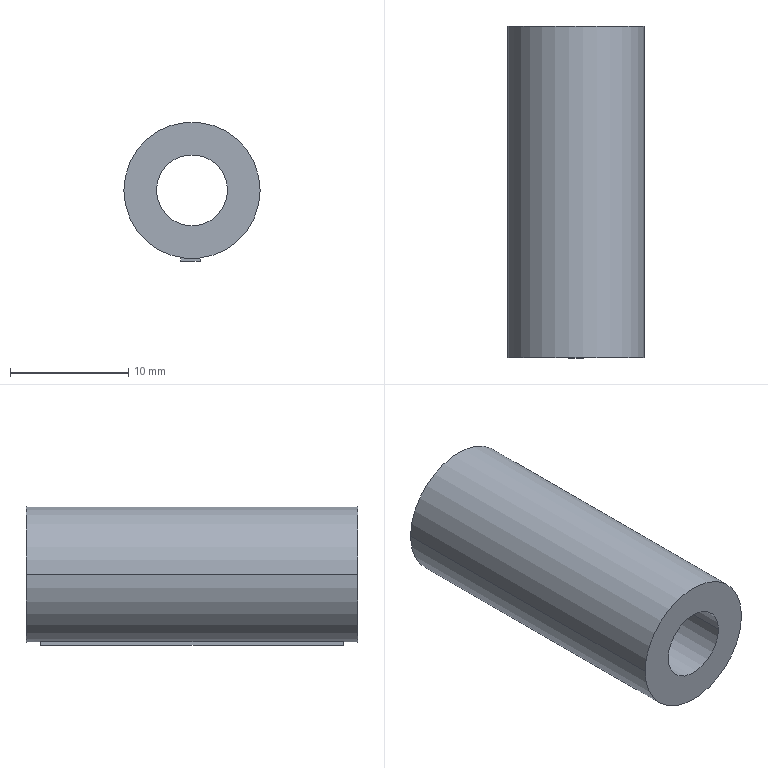Component | SolidWorks | Hinge1-1 | 1 solid | 11 faces | box 11.5 x 28 x 11.75 mm | volume 2128 mm3 | plane 7 | cylinder 4 | commonest cylinder face diameters 6 x2 11.5 x2
build123d program:
from build123d import *

# Parameters (mm, degrees)
SKETCH1_R                = 5.75
SKETCH1_R_2              = 3
BOSS_EXTRUDE1_DEPTH      = 14
BOSS_EXTRUDE2_REACH      = 23.728
BOSS_EXTRUDE2_END_RADIUS = 5.75
SKETCH2_W                = 1.644
SKETCH2_H                = 25.571


with BuildPart() as part:
    # Sketch1 → Boss-Extrude1 (new, symmetric)
    with BuildSketch(Plane(origin=(0, 0, 0), x_dir=(1, 0, 0), z_dir=(0, 1, 0))):
        with Locations(Location((6, -6, 0), (0, 0, 270))):
            Circle(SKETCH1_R)
        with Locations(Location((6, -6, 0), (0, 0, 270))):
            Circle(SKETCH1_R_2, mode=Mode.SUBTRACT)
    extrude(amount=BOSS_EXTRUDE1_DEPTH, both=True)

    # Boss-Extrude2: up to this cylinder (the profile starts outside it)
    boss_extrude2_end = Plane(origin=(6, 0, 6), z_dir=(0, -1, 0)) * Cylinder(BOSS_EXTRUDE2_END_RADIUS, 59.956, mode=Mode.PRIVATE)
    # Sketch2 → Boss-Extrude2 (add, up to the surface)
    with BuildSketch(Plane(origin=(0, 0, 0), x_dir=(0, 0, -1), z_dir=(1, 0, 0)), mode=Mode.PRIVATE) as boss_extrude2_sk1:
        with Locations((-6.137, 0)):
            Rectangle(SKETCH2_W, SKETCH2_H)
    boss_extrude2_tool1 = extrude(boss_extrude2_sk1.sketch, amount=BOSS_EXTRUDE2_REACH, mode=Mode.PRIVATE) - boss_extrude2_end
    add(boss_extrude2_tool1.solids().sort_by_distance((0, 0, 6.137))[0])


solid = part.part

# Placed as in the assembly
solid = solid.moved(Location((229.391, -336.131, 906.387), (0, -90, 0)))
STEP:
#1=COLOUR_RGB('',0.7922,0.8196,0.9333);
#2=FILL_AREA_STYLE_COLOUR('',#1);
#3=FILL_AREA_STYLE('',(#2));
#4=SURFACE_STYLE_FILL_AREA(#3);
#5=SURFACE_SIDE_STYLE('',(#4));
#6=SURFACE_STYLE_USAGE(.BOTH.,#5);
#7=PRESENTATION_STYLE_ASSIGNMENT((#6));
#8=CARTESIAN_POINT('',(8.913,-12.682,35.921));
#9=VERTEX_POINT('',#8);
#10=CARTESIAN_POINT('',(8.677,-12.682,35.921));
#11=VERTEX_POINT('',#10);
#12=CARTESIAN_POINT('',(8.795,-12.682,35.921));
#13=DIRECTION('',(0.,1.,0.));
#14=DIRECTION('',(-1.,0.,0.));
#15=AXIS2_PLACEMENT_3D('',#12,#13,#14);
#16=CIRCLE('',#15,0.1181);
#17=EDGE_CURVE('',#9,#11,#16,.T.);
#18=ORIENTED_EDGE('',*,*,#17,.T.);
#19=CARTESIAN_POINT('',(8.677,-13.785,35.921));
#20=VERTEX_POINT('',#19);
#21=CARTESIAN_POINT('',(8.677,-12.682,35.921));
#22=DIRECTION('',(0.,-1.,0.));
#23=VECTOR('',#22,39.37);
#24=LINE('',#21,#23);
#25=EDGE_CURVE('',#11,#20,#24,.T.);
#26=ORIENTED_EDGE('',*,*,#25,.T.);
#27=CARTESIAN_POINT('',(8.913,-13.785,35.921));
#28=VERTEX_POINT('',#27);
#29=CARTESIAN_POINT('',(8.795,-13.785,35.921));
#30=DIRECTION('',(0.,1.,0.));
#31=DIRECTION('',(-1.,0.,0.));
#32=AXIS2_PLACEMENT_3D('',#29,#30,#31);
#33=CIRCLE('',#32,0.1181);
#34=EDGE_CURVE('',#28,#20,#33,.T.);
#35=ORIENTED_EDGE('',*,*,#34,.F.);
#36=CARTESIAN_POINT('',(8.913,-12.682,35.921));
#37=DIRECTION('',(0.,-1.,0.));
#38=VECTOR('',#37,39.37);
#39=LINE('',#36,#38);
#40=EDGE_CURVE('',#9,#28,#39,.T.);
#41=ORIENTED_EDGE('',*,*,#40,.F.);
#42=EDGE_LOOP('',(#18,#26,#35,#41));
#43=FACE_OUTER_BOUND('',#42,.T.);
#44=CARTESIAN_POINT('',(8.795,-12.682,35.921));
#45=DIRECTION('',(0.,-1.,0.));
#46=DIRECTION('',(1.,0.,0.));
#47=AXIS2_PLACEMENT_3D('',#44,#45,#46);
#48=CYLINDRICAL_SURFACE('',#47,0.1181);
#49=ADVANCED_FACE('',(#43),#48,.F.);
#50=CARTESIAN_POINT('',(8.569,-12.682,35.921));
#51=VERTEX_POINT('',#50);
#52=CARTESIAN_POINT('',(9.021,-12.682,35.921));
#53=VERTEX_POINT('',#52);
#54=CARTESIAN_POINT('',(8.795,-12.682,35.921));
#55=DIRECTION('',(0.,1.,0.));
#56=DIRECTION('',(-1.,0.,0.));
#57=AXIS2_PLACEMENT_3D('',#54,#55,#56);
#58=CIRCLE('',#57,0.2264);
#59=EDGE_CURVE('',#51,#53,#58,.T.);
#60=ORIENTED_EDGE('',*,*,#59,.F.);
#61=CARTESIAN_POINT('',(8.569,-13.785,35.921));
#62=VERTEX_POINT('',#61);
#63=CARTESIAN_POINT('',(8.569,-12.682,35.921));
#64=DIRECTION('',(0.,-1.,0.));
#65=VECTOR('',#64,39.37);
#66=LINE('',#63,#65);
#67=EDGE_CURVE('',#51,#62,#66,.T.);
#68=ORIENTED_EDGE('',*,*,#67,.T.);
#69=CARTESIAN_POINT('',(9.021,-13.785,35.921));
#70=VERTEX_POINT('',#69);
#71=CARTESIAN_POINT('',(8.795,-13.785,35.921));
#72=DIRECTION('',(0.,1.,0.));
#73=DIRECTION('',(-1.,0.,0.));
#74=AXIS2_PLACEMENT_3D('',#71,#72,#73);
#75=CIRCLE('',#74,0.2264);
#76=EDGE_CURVE('',#62,#70,#75,.T.);
#77=ORIENTED_EDGE('',*,*,#76,.T.);
#78=CARTESIAN_POINT('',(9.021,-12.682,35.921));
#79=DIRECTION('',(0.,-1.,0.));
#80=VECTOR('',#79,39.37);
#81=LINE('',#78,#80);
#82=EDGE_CURVE('',#53,#70,#81,.T.);
#83=ORIENTED_EDGE('',*,*,#82,.F.);
#84=EDGE_LOOP('',(#60,#68,#77,#83));
#85=FACE_OUTER_BOUND('',#84,.T.);
#86=CARTESIAN_POINT('',(8.795,-12.682,35.921));
#87=DIRECTION('',(0.,-1.,0.));
#88=DIRECTION('',(1.,0.,0.));
#89=AXIS2_PLACEMENT_3D('',#86,#87,#88);
#90=CYLINDRICAL_SURFACE('',#89,0.2264);
#91=ADVANCED_FACE('',(#85),#90,.T.);
#92=ORIENTED_EDGE('',*,*,#67,.F.);
#93=CARTESIAN_POINT('',(8.795,-12.682,35.921));
#94=DIRECTION('',(0.,1.,0.));
#95=DIRECTION('',(-1.,0.,0.));
#96=AXIS2_PLACEMENT_3D('',#93,#94,#95);
#97=CIRCLE('',#96,0.2264);
#98=EDGE_CURVE('',#53,#51,#97,.T.);
#99=ORIENTED_EDGE('',*,*,#98,.F.);
#100=ORIENTED_EDGE('',*,*,#82,.T.);
#101=CARTESIAN_POINT('',(8.795,-13.785,35.921));
#102=DIRECTION('',(0.,1.,0.));
#103=DIRECTION('',(-1.,0.,0.));
#104=AXIS2_PLACEMENT_3D('',#101,#102,#103);
#105=CIRCLE('',#104,0.2264);
#106=EDGE_CURVE('',#70,#62,#105,.T.);
#107=ORIENTED_EDGE('',*,*,#106,.T.);
#108=EDGE_LOOP('',(#92,#99,#100,#107));
#109=FACE_OUTER_BOUND('',#108,.T.);
#110=CARTESIAN_POINT('',(8.757,-12.73,35.698));
#111=VERTEX_POINT('',#110);
#112=CARTESIAN_POINT('',(8.757,-13.737,35.698));
#113=VERTEX_POINT('',#112);
#114=CARTESIAN_POINT('',(8.757,-12.682,35.698));
#115=DIRECTION('',(0.,-1.,0.));
#116=VECTOR('',#115,39.37);
#117=LINE('',#114,#116);
#118=EDGE_CURVE('',#111,#113,#117,.T.);
#119=ORIENTED_EDGE('',*,*,#118,.T.);
#120=CARTESIAN_POINT('',(8.822,-13.737,35.696));
#121=VERTEX_POINT('',#120);
#122=CARTESIAN_POINT('',(8.795,-13.737,35.921));
#123=DIRECTION('',(0.,-1.,0.));
#124=DIRECTION('',(-1.,0.,0.));
#125=AXIS2_PLACEMENT_3D('',#122,#123,#124);
#126=CIRCLE('',#125,0.2264);
#127=EDGE_CURVE('',#113,#121,#126,.T.);
#128=ORIENTED_EDGE('',*,*,#127,.T.);
#129=CARTESIAN_POINT('',(8.822,-12.73,35.696));
#130=VERTEX_POINT('',#129);
#131=CARTESIAN_POINT('',(8.822,-12.682,35.696));
#132=DIRECTION('',(0.,1.,0.));
#133=VECTOR('',#132,39.37);
#134=LINE('',#131,#133);
#135=EDGE_CURVE('',#121,#130,#134,.T.);
#136=ORIENTED_EDGE('',*,*,#135,.T.);
#137=CARTESIAN_POINT('',(8.795,-12.73,35.921));
#138=DIRECTION('',(0.,1.,0.));
#139=DIRECTION('',(1.,0.,0.));
#140=AXIS2_PLACEMENT_3D('',#137,#138,#139);
#141=CIRCLE('',#140,0.2264);
#142=EDGE_CURVE('',#130,#111,#141,.T.);
#143=ORIENTED_EDGE('',*,*,#142,.T.);
#144=EDGE_LOOP('',(#119,#128,#136,#143));
#145=FACE_BOUND('',#144,.T.);
#146=CARTESIAN_POINT('',(8.795,-12.682,35.921));
#147=DIRECTION('',(0.,-1.,0.));
#148=DIRECTION('',(1.,0.,0.));
#149=AXIS2_PLACEMENT_3D('',#146,#147,#148);
#150=CYLINDRICAL_SURFACE('',#149,0.2264);
#151=ADVANCED_FACE('',(#109,#145),#150,.T.);
#152=ORIENTED_EDGE('',*,*,#98,.T.);
#153=ORIENTED_EDGE('',*,*,#59,.T.);
#154=EDGE_LOOP('',(#152,#153));
#155=FACE_OUTER_BOUND('',#154,.T.);
#156=ORIENTED_EDGE('',*,*,#17,.F.);
#157=CARTESIAN_POINT('',(8.795,-12.682,35.921));
#158=DIRECTION('',(0.,1.,0.));
#159=DIRECTION('',(-1.,0.,0.));
#160=AXIS2_PLACEMENT_3D('',#157,#158,#159);
#161=CIRCLE('',#160,0.1181);
#162=EDGE_CURVE('',#11,#9,#161,.T.);
#163=ORIENTED_EDGE('',*,*,#162,.F.);
#164=EDGE_LOOP('',(#156,#163));
#165=FACE_BOUND('',#164,.T.);
#166=CARTESIAN_POINT('',(8.795,-12.682,35.921));
#167=DIRECTION('',(0.,1.,0.));
#168=DIRECTION('',(-1.,0.,-0.));
#169=AXIS2_PLACEMENT_3D('',#166,#167,#168);
#170=PLANE('',#169);
#171=ADVANCED_FACE('',(#155,#165),#170,.T.);
#172=ORIENTED_EDGE('',*,*,#106,.F.);
#173=ORIENTED_EDGE('',*,*,#76,.F.);
#174=EDGE_LOOP('',(#172,#173));
#175=FACE_OUTER_BOUND('',#174,.T.);
#176=ORIENTED_EDGE('',*,*,#34,.T.);
#177=CARTESIAN_POINT('',(8.795,-13.785,35.921));
#178=DIRECTION('',(0.,1.,0.));
#179=DIRECTION('',(-1.,0.,0.));
#180=AXIS2_PLACEMENT_3D('',#177,#178,#179);
#181=CIRCLE('',#180,0.1181);
#182=EDGE_CURVE('',#20,#28,#181,.T.);
#183=ORIENTED_EDGE('',*,*,#182,.T.);
#184=EDGE_LOOP('',(#176,#183));
#185=FACE_BOUND('',#184,.T.);
#186=CARTESIAN_POINT('',(8.795,-13.785,35.921));
#187=DIRECTION('',(0.,1.,0.));
#188=DIRECTION('',(-1.,0.,-0.));
#189=AXIS2_PLACEMENT_3D('',#186,#187,#188);
#190=PLANE('',#189);
#191=ADVANCED_FACE('',(#175,#185),#190,.F.);
#192=ORIENTED_EDGE('',*,*,#25,.F.);
#193=ORIENTED_EDGE('',*,*,#162,.T.);
#194=ORIENTED_EDGE('',*,*,#40,.T.);
#195=ORIENTED_EDGE('',*,*,#182,.F.);
#196=EDGE_LOOP('',(#192,#193,#194,#195));
#197=FACE_OUTER_BOUND('',#196,.T.);
#198=CARTESIAN_POINT('',(8.795,-12.682,35.921));
#199=DIRECTION('',(0.,-1.,0.));
#200=DIRECTION('',(1.,0.,0.));
#201=AXIS2_PLACEMENT_3D('',#198,#199,#200);
#202=CYLINDRICAL_SURFACE('',#201,0.1181);
#203=ADVANCED_FACE('',(#197),#202,.F.);
#204=CARTESIAN_POINT('',(8.757,-12.73,35.685));
#205=VERTEX_POINT('',#204);
#206=CARTESIAN_POINT('',(8.757,-13.737,35.685));
#207=VERTEX_POINT('',#206);
#208=CARTESIAN_POINT('',(8.757,-13.737,35.685));
#209=DIRECTION('',(0.,-1.,0.));
#210=VECTOR('',#209,39.37);
#211=LINE('',#208,#210);
#212=EDGE_CURVE('',#205,#207,#211,.T.);
#213=ORIENTED_EDGE('',*,*,#212,.F.);
#214=CARTESIAN_POINT('',(8.822,-12.73,35.685));
#215=VERTEX_POINT('',#214);
#216=CARTESIAN_POINT('',(8.822,-12.73,35.685));
#217=DIRECTION('',(-1.,0.,-0.));
#218=VECTOR('',#217,39.37);
#219=LINE('',#216,#218);
#220=EDGE_CURVE('',#215,#205,#219,.T.);
#221=ORIENTED_EDGE('',*,*,#220,.F.);
#222=CARTESIAN_POINT('',(8.822,-13.737,35.685));
#223=VERTEX_POINT('',#222);
#224=CARTESIAN_POINT('',(8.822,-13.737,35.685));
#225=DIRECTION('',(0.,1.,0.));
#226=VECTOR('',#225,39.37);
#227=LINE('',#224,#226);
#228=EDGE_CURVE('',#223,#215,#227,.T.);
#229=ORIENTED_EDGE('',*,*,#228,.F.);
#230=CARTESIAN_POINT('',(8.822,-13.737,35.685));
#231=DIRECTION('',(1.,0.,0.));
#232=VECTOR('',#231,39.37);
#233=LINE('',#230,#232);
#234=EDGE_CURVE('',#207,#223,#233,.T.);
#235=ORIENTED_EDGE('',*,*,#234,.F.);
#236=EDGE_LOOP('',(#213,#221,#229,#235));
#237=FACE_OUTER_BOUND('',#236,.T.);
#238=CARTESIAN_POINT('',(9.031,-13.234,35.685));
#239=DIRECTION('',(-0.,0.,1.));
#240=DIRECTION('',(1.,0.,0.));
#241=AXIS2_PLACEMENT_3D('',#238,#239,#240);
#242=PLANE('',#241);
#243=ADVANCED_FACE('',(#237),#242,.F.);
#244=ORIENTED_EDGE('',*,*,#142,.F.);
#245=CARTESIAN_POINT('',(8.822,-12.73,19720.724));
#246=DIRECTION('',(0.,0.,-1.));
#247=VECTOR('',#246,39.37);
#248=LINE('',#245,#247);
#249=EDGE_CURVE('',#130,#215,#248,.T.);
#250=ORIENTED_EDGE('',*,*,#249,.T.);
#251=ORIENTED_EDGE('',*,*,#220,.T.);
#252=CARTESIAN_POINT('',(8.757,-12.73,19720.724));
#253=DIRECTION('',(0.,0.,-1.));
#254=VECTOR('',#253,39.37);
#255=LINE('',#252,#254);
#256=EDGE_CURVE('',#111,#205,#255,.T.);
#257=ORIENTED_EDGE('',*,*,#256,.F.);
#258=EDGE_LOOP('',(#244,#250,#251,#257));
#259=FACE_OUTER_BOUND('',#258,.T.);
#260=CARTESIAN_POINT('',(8.822,-12.73,19720.724));
#261=DIRECTION('',(0.,-1.,0.));
#262=DIRECTION('',(1.,0.,0.));
#263=AXIS2_PLACEMENT_3D('',#260,#261,#262);
#264=PLANE('',#263);
#265=ADVANCED_FACE('',(#259),#264,.F.);
#266=ORIENTED_EDGE('',*,*,#135,.F.);
#267=CARTESIAN_POINT('',(8.822,-13.737,19720.724));
#268=DIRECTION('',(0.,0.,-1.));
#269=VECTOR('',#268,39.37);
#270=LINE('',#267,#269);
#271=EDGE_CURVE('',#121,#223,#270,.T.);
#272=ORIENTED_EDGE('',*,*,#271,.T.);
#273=ORIENTED_EDGE('',*,*,#228,.T.);
#274=ORIENTED_EDGE('',*,*,#249,.F.);
#275=EDGE_LOOP('',(#266,#272,#273,#274));
#276=FACE_OUTER_BOUND('',#275,.T.);
#277=CARTESIAN_POINT('',(8.822,-13.737,19720.724));
#278=DIRECTION('',(-1.,0.,-0.));
#279=DIRECTION('',(-0.,0.,1.));
#280=AXIS2_PLACEMENT_3D('',#277,#278,#279);
#281=PLANE('',#280);
#282=ADVANCED_FACE('',(#276),#281,.F.);
#283=ORIENTED_EDGE('',*,*,#127,.F.);
#284=CARTESIAN_POINT('',(8.757,-13.737,19720.724));
#285=DIRECTION('',(0.,0.,-1.));
#286=VECTOR('',#285,39.37);
#287=LINE('',#284,#286);
#288=EDGE_CURVE('',#113,#207,#287,.T.);
#289=ORIENTED_EDGE('',*,*,#288,.T.);
#290=ORIENTED_EDGE('',*,*,#234,.T.);
#291=ORIENTED_EDGE('',*,*,#271,.F.);
#292=EDGE_LOOP('',(#283,#289,#290,#291));
#293=FACE_OUTER_BOUND('',#292,.T.);
#294=CARTESIAN_POINT('',(8.822,-13.737,19720.724));
#295=DIRECTION('',(0.,1.,0.));
#296=DIRECTION('',(-1.,0.,-0.));
#297=AXIS2_PLACEMENT_3D('',#294,#295,#296);
#298=PLANE('',#297);
#299=ADVANCED_FACE('',(#293),#298,.F.);
#300=ORIENTED_EDGE('',*,*,#118,.F.);
#301=ORIENTED_EDGE('',*,*,#256,.T.);
#302=ORIENTED_EDGE('',*,*,#212,.T.);
#303=ORIENTED_EDGE('',*,*,#288,.F.);
#304=EDGE_LOOP('',(#300,#301,#302,#303));
#305=FACE_OUTER_BOUND('',#304,.T.);
#306=CARTESIAN_POINT('',(8.757,-13.737,19720.724));
#307=DIRECTION('',(1.,0.,0.));
#308=DIRECTION('',(0.,0.,-1.));
#309=AXIS2_PLACEMENT_3D('',#306,#307,#308);
#310=PLANE('',#309);
#311=ADVANCED_FACE('',(#305),#310,.F.);
#312=CLOSED_SHELL('',(#49,#91,#151,#171,#191,#203,#243,#265,#282,#299,#311));
#313=MANIFOLD_SOLID_BREP('',#312);
#314=STYLED_ITEM('',(#7),#313);
#315=PRESENTATION_LAYER_ASSIGNMENT('','',(#314));
#316=(LENGTH_UNIT()NAMED_UNIT(*)SI_UNIT($,.METRE.));
#317=LENGTH_MEASURE_WITH_UNIT(LENGTH_MEASURE(0.0254),#316);
#318=DIMENSIONAL_EXPONENTS(1.,0.,0.,0.,0.,0.,0.);
#319=(CONVERSION_BASED_UNIT('',#317)LENGTH_UNIT()NAMED_UNIT(#318));
#320=UNCERTAINTY_MEASURE_WITH_UNIT(LENGTH_MEASURE(0.00001),#319,'','');
#321=(NAMED_UNIT(*)PLANE_ANGLE_UNIT()SI_UNIT($,.RADIAN.));
#322=(NAMED_UNIT(*)SI_UNIT($,.STERADIAN.)SOLID_ANGLE_UNIT());
#323=(GEOMETRIC_REPRESENTATION_CONTEXT(3)GLOBAL_UNCERTAINTY_ASSIGNED_CONTEXT((#320))GLOBAL_UNIT_ASSIGNED_CONTEXT((#319,#321,#322))REPRESENTATION_CONTEXT('',''));
#324=MECHANICAL_DESIGN_GEOMETRIC_PRESENTATION_REPRESENTATION('',(#314),#323);
#325=CARTESIAN_POINT('',(0.,0.,0.));
#326=DIRECTION('',(0.,0.,1.));
#327=DIRECTION('',(1.,0.,0.));
#328=AXIS2_PLACEMENT_3D('',#325,#326,#327);
#329=(LENGTH_UNIT()NAMED_UNIT(*)SI_UNIT($,.METRE.));
#330=LENGTH_MEASURE_WITH_UNIT(LENGTH_MEASURE(0.0254),#329);
#331=DIMENSIONAL_EXPONENTS(1.,0.,0.,0.,0.,0.,0.);
#332=(CONVERSION_BASED_UNIT('',#330)LENGTH_UNIT()NAMED_UNIT(#331));
#333=UNCERTAINTY_MEASURE_WITH_UNIT(LENGTH_MEASURE(0.00001),#332,'','');
#334=(NAMED_UNIT(*)PLANE_ANGLE_UNIT()SI_UNIT($,.RADIAN.));
#335=(NAMED_UNIT(*)SI_UNIT($,.STERADIAN.)SOLID_ANGLE_UNIT());
#336=(GEOMETRIC_REPRESENTATION_CONTEXT(3)GLOBAL_UNCERTAINTY_ASSIGNED_CONTEXT((#333))GLOBAL_UNIT_ASSIGNED_CONTEXT((#332,#334,#335))REPRESENTATION_CONTEXT('',''));
#337=ADVANCED_BREP_SHAPE_REPRESENTATION('',(#313,#328),#336);